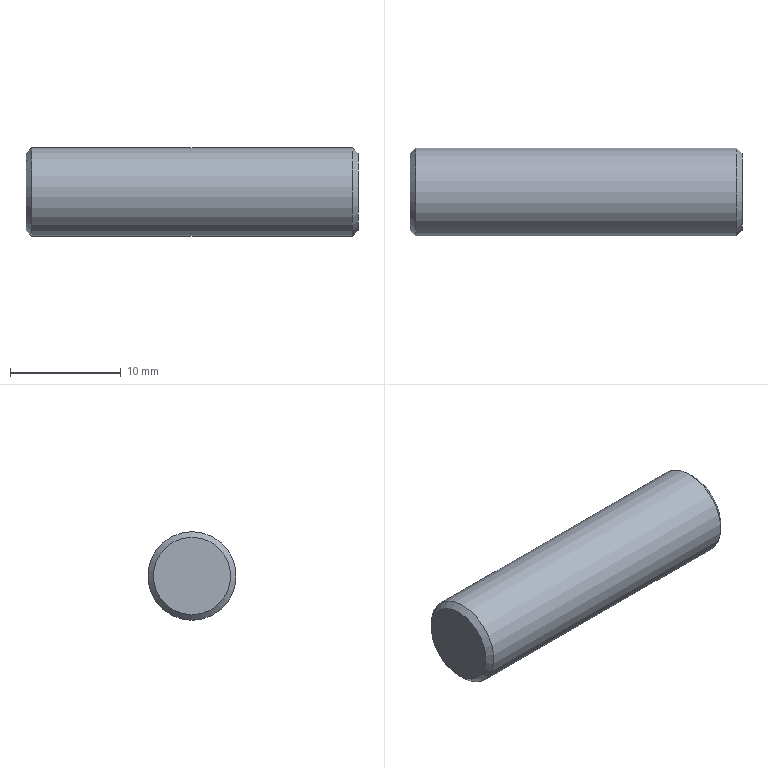Component | NX | DOWEL_PIN_8X30 | 1 solid | 5 faces | box 30 x 8 x 8 mm | volume 1502 mm3 | plane 2 | cone 2 | cylinder 1 | commonest cylinder face diameters 8 x1
STEP:
#1=CARTESIAN_POINT('',(0.,0.,0.));
#2=DIRECTION('',(0.,0.,1.));
#3=DIRECTION('',(1.,0.,0.));
#4=AXIS2_PLACEMENT_3D('',#1,#2,#3);
#5=CARTESIAN_POINT('',(59.511,45.372,16.));
#6=VERTEX_POINT('',#5);
#7=CARTESIAN_POINT('',(59.511,45.372,20.));
#8=DIRECTION('',(-1.,0.,0.));
#9=DIRECTION('',(0.,0.,-1.));
#10=AXIS2_PLACEMENT_3D('',#7,#8,#9);
#11=CIRCLE('',#10,4.);
#12=CARTESIAN_POINT('',(50.011,45.372,20.));
#13=DIRECTION('',(-1.,0.,0.));
#14=DIRECTION('',(0.,0.,1.));
#15=AXIS2_PLACEMENT_3D('',#12,#13,#14);
#16=CYLINDRICAL_SURFACE('',#15,4.);
#17=CARTESIAN_POINT('',(3.142,-9.5));
#18=DIRECTION('',(1.,0.));
#19=VECTOR('',#18,1.);
#20=LINE('',#17,#19);
#21=(GEOMETRIC_REPRESENTATION_CONTEXT(2)PARAMETRIC_REPRESENTATION_CONTEXT()REPRESENTATION_CONTEXT('',''));
#22=DEFINITIONAL_REPRESENTATION('',(#20),#21);
#23=PCURVE('',#16,#22);
#24=CARTESIAN_POINT('',(60.011,45.372,20.));
#25=DIRECTION('',(-1.,0.,0.));
#26=DIRECTION('',(0.,0.,1.));
#27=AXIS2_PLACEMENT_3D('',#24,#25,#26);
#28=CONICAL_SURFACE('',#27,3.5,0.7854);
#29=CARTESIAN_POINT('',(3.142,0.5));
#30=DIRECTION('',(1.,0.));
#31=VECTOR('',#30,1.);
#32=LINE('',#29,#31);
#33=(GEOMETRIC_REPRESENTATION_CONTEXT(2)PARAMETRIC_REPRESENTATION_CONTEXT()REPRESENTATION_CONTEXT('',''));
#34=DEFINITIONAL_REPRESENTATION('',(#32),#33);
#35=PCURVE('',#28,#34);
#36=SURFACE_CURVE('',#11,(#23,#35),.PCURVE_S1.);
#37=EDGE_CURVE('',#6,#6,#36,.T.);
#38=ORIENTED_EDGE('',*,*,#37,.T.);
#39=CARTESIAN_POINT('',(30.511,45.372,16.));
#40=VERTEX_POINT('',#39);
#41=CARTESIAN_POINT('',(59.511,45.372,16.));
#42=CARTESIAN_POINT('',(30.511,45.372,16.));
#43=B_SPLINE_CURVE_WITH_KNOTS('',1,(#41,#42),.UNSPECIFIED.,.F.,.F.,(2,2),(-9.5,19.5),.PIECEWISE_BEZIER_KNOTS.);
#44=CARTESIAN_POINT('',(9.425,0.));
#45=DIRECTION('',(0.,1.));
#46=VECTOR('',#45,1.);
#47=LINE('',#44,#46);
#48=(GEOMETRIC_REPRESENTATION_CONTEXT(2)PARAMETRIC_REPRESENTATION_CONTEXT()REPRESENTATION_CONTEXT('',''));
#49=DEFINITIONAL_REPRESENTATION('',(#47),#48);
#50=PCURVE('',#16,#49);
#51=CARTESIAN_POINT('',(3.142,0.));
#52=DIRECTION('',(0.,1.));
#53=VECTOR('',#52,1.);
#54=LINE('',#51,#53);
#55=(GEOMETRIC_REPRESENTATION_CONTEXT(2)PARAMETRIC_REPRESENTATION_CONTEXT()REPRESENTATION_CONTEXT('',''));
#56=DEFINITIONAL_REPRESENTATION('',(#54),#55);
#57=PCURVE('',#16,#56);
#58=SEAM_CURVE('',#43,(#50,#57),.PCURVE_S1.);
#59=EDGE_CURVE('',#6,#40,#58,.T.);
#60=ORIENTED_EDGE('',*,*,#59,.T.);
#61=CARTESIAN_POINT('',(30.511,45.372,20.));
#62=DIRECTION('',(1.,0.,0.));
#63=DIRECTION('',(0.,0.,-1.));
#64=AXIS2_PLACEMENT_3D('',#61,#62,#63);
#65=CIRCLE('',#64,4.);
#66=CARTESIAN_POINT('',(9.425,19.5));
#67=DIRECTION('',(-1.,0.));
#68=VECTOR('',#67,1.);
#69=LINE('',#66,#68);
#70=(GEOMETRIC_REPRESENTATION_CONTEXT(2)PARAMETRIC_REPRESENTATION_CONTEXT()REPRESENTATION_CONTEXT('',''));
#71=DEFINITIONAL_REPRESENTATION('',(#69),#70);
#72=PCURVE('',#16,#71);
#73=CARTESIAN_POINT('',(30.511,45.372,20.));
#74=DIRECTION('',(1.,0.,0.));
#75=DIRECTION('',(0.,0.,-1.));
#76=AXIS2_PLACEMENT_3D('',#73,#74,#75);
#77=CONICAL_SURFACE('',#76,4.,0.7854);
#78=CARTESIAN_POINT('',(0.,0.));
#79=DIRECTION('',(1.,0.));
#80=VECTOR('',#79,1.);
#81=LINE('',#78,#80);
#82=(GEOMETRIC_REPRESENTATION_CONTEXT(2)PARAMETRIC_REPRESENTATION_CONTEXT()REPRESENTATION_CONTEXT('',''));
#83=DEFINITIONAL_REPRESENTATION('',(#81),#82);
#84=PCURVE('',#77,#83);
#85=SURFACE_CURVE('',#65,(#72,#84),.PCURVE_S1.);
#86=EDGE_CURVE('',#40,#40,#85,.T.);
#87=ORIENTED_EDGE('',*,*,#86,.T.);
#88=ORIENTED_EDGE('',*,*,#59,.F.);
#89=EDGE_LOOP('',(#38,#60,#87,#88));
#90=FACE_BOUND('',#89,.T.);
#91=ADVANCED_FACE('',(#90),#16,.T.);
#92=CARTESIAN_POINT('',(60.011,45.372,16.5));
#93=VERTEX_POINT('',#92);
#94=CARTESIAN_POINT('',(60.011,45.372,20.));
#95=DIRECTION('',(1.,0.,0.));
#96=DIRECTION('',(0.,0.,-1.));
#97=AXIS2_PLACEMENT_3D('',#94,#95,#96);
#98=CIRCLE('',#97,3.5);
#99=CARTESIAN_POINT('',(60.011,45.372,20.));
#100=DIRECTION('',(1.,0.,0.));
#101=DIRECTION('',(0.,0.,-1.));
#102=AXIS2_PLACEMENT_3D('',#99,#100,#101);
#103=PLANE('',#102);
#104=CARTESIAN_POINT('',(0.,0.));
#105=DIRECTION('',(1.,0.));
#106=AXIS2_PLACEMENT_2D('',#104,#105);
#107=CIRCLE('',#106,3.5);
#108=(GEOMETRIC_REPRESENTATION_CONTEXT(2)PARAMETRIC_REPRESENTATION_CONTEXT()REPRESENTATION_CONTEXT('',''));
#109=DEFINITIONAL_REPRESENTATION('',(#107),#108);
#110=PCURVE('',#103,#109);
#111=CARTESIAN_POINT('',(9.425,0.));
#112=DIRECTION('',(-1.,0.));
#113=VECTOR('',#112,1.);
#114=LINE('',#111,#113);
#115=(GEOMETRIC_REPRESENTATION_CONTEXT(2)PARAMETRIC_REPRESENTATION_CONTEXT()REPRESENTATION_CONTEXT('',''));
#116=DEFINITIONAL_REPRESENTATION('',(#114),#115);
#117=PCURVE('',#28,#116);
#118=SURFACE_CURVE('',#98,(#110,#117),.PCURVE_S1.);
#119=EDGE_CURVE('',#93,#93,#118,.T.);
#120=ORIENTED_EDGE('',*,*,#119,.T.);
#121=EDGE_LOOP('',(#120));
#122=FACE_BOUND('',#121,.T.);
#123=ADVANCED_FACE('',(#122),#103,.T.);
#124=CARTESIAN_POINT('',(30.011,45.372,16.5));
#125=VERTEX_POINT('',#124);
#126=CARTESIAN_POINT('',(30.011,45.372,20.));
#127=DIRECTION('',(-1.,0.,0.));
#128=DIRECTION('',(0.,0.,-1.));
#129=AXIS2_PLACEMENT_3D('',#126,#127,#128);
#130=CIRCLE('',#129,3.5);
#131=CARTESIAN_POINT('',(30.011,45.372,20.));
#132=DIRECTION('',(1.,0.,0.));
#133=DIRECTION('',(0.,0.,-1.));
#134=AXIS2_PLACEMENT_3D('',#131,#132,#133);
#135=PLANE('',#134);
#136=CARTESIAN_POINT('',(3.5,0.));
#137=CARTESIAN_POINT('',(3.5,-6.062));
#138=CARTESIAN_POINT('',(-1.75,-3.031));
#139=CARTESIAN_POINT('',(-7.,-0.));
#140=CARTESIAN_POINT('',(-1.75,3.031));
#141=CARTESIAN_POINT('',(3.5,6.062));
#142=CARTESIAN_POINT('',(3.5,0.));
#143=(BOUNDED_CURVE()B_SPLINE_CURVE(2,(#136,#137,#138,#139,#140,#141,#142),.UNSPECIFIED.,.T.,.F.)B_SPLINE_CURVE_WITH_KNOTS((1,2,2,2,2,1),(-2.094,0.,2.094,4.189,6.283,8.378),.UNSPECIFIED.)CURVE()GEOMETRIC_REPRESENTATION_ITEM()RATIONAL_B_SPLINE_CURVE((1.,0.5,1.,0.5,1.,0.5,1.))REPRESENTATION_ITEM(''));
#144=(GEOMETRIC_REPRESENTATION_CONTEXT(2)PARAMETRIC_REPRESENTATION_CONTEXT()REPRESENTATION_CONTEXT('',''));
#145=DEFINITIONAL_REPRESENTATION('',(#143),#144);
#146=PCURVE('',#135,#145);
#147=CARTESIAN_POINT('',(6.283,-0.5));
#148=DIRECTION('',(-1.,0.));
#149=VECTOR('',#148,1.);
#150=LINE('',#147,#149);
#151=(GEOMETRIC_REPRESENTATION_CONTEXT(2)PARAMETRIC_REPRESENTATION_CONTEXT()REPRESENTATION_CONTEXT('',''));
#152=DEFINITIONAL_REPRESENTATION('',(#150),#151);
#153=PCURVE('',#77,#152);
#154=SURFACE_CURVE('',#130,(#146,#153),.PCURVE_S1.);
#155=EDGE_CURVE('',#125,#125,#154,.T.);
#156=ORIENTED_EDGE('',*,*,#155,.T.);
#157=EDGE_LOOP('',(#156));
#158=FACE_BOUND('',#157,.T.);
#159=ADVANCED_FACE('',(#158),#135,.F.);
#160=ORIENTED_EDGE('',*,*,#37,.F.);
#161=CARTESIAN_POINT('',(60.011,45.372,16.5));
#162=CARTESIAN_POINT('',(59.511,45.372,16.));
#163=B_SPLINE_CURVE_WITH_KNOTS('',1,(#161,#162),.UNSPECIFIED.,.F.,.F.,(2,2),(0.,0.7071),.PIECEWISE_BEZIER_KNOTS.);
#164=CARTESIAN_POINT('',(3.142,0.));
#165=DIRECTION('',(0.,1.));
#166=VECTOR('',#165,1.);
#167=LINE('',#164,#166);
#168=(GEOMETRIC_REPRESENTATION_CONTEXT(2)PARAMETRIC_REPRESENTATION_CONTEXT()REPRESENTATION_CONTEXT('',''));
#169=DEFINITIONAL_REPRESENTATION('',(#167),#168);
#170=PCURVE('',#28,#169);
#171=CARTESIAN_POINT('',(9.425,0.));
#172=DIRECTION('',(0.,1.));
#173=VECTOR('',#172,1.);
#174=LINE('',#171,#173);
#175=(GEOMETRIC_REPRESENTATION_CONTEXT(2)PARAMETRIC_REPRESENTATION_CONTEXT()REPRESENTATION_CONTEXT('',''));
#176=DEFINITIONAL_REPRESENTATION('',(#174),#175);
#177=PCURVE('',#28,#176);
#178=SEAM_CURVE('',#163,(#170,#177),.PCURVE_S1.);
#179=EDGE_CURVE('',#93,#6,#178,.T.);
#180=ORIENTED_EDGE('',*,*,#179,.F.);
#181=ORIENTED_EDGE('',*,*,#119,.F.);
#182=ORIENTED_EDGE('',*,*,#179,.T.);
#183=EDGE_LOOP('',(#160,#180,#181,#182));
#184=FACE_BOUND('',#183,.T.);
#185=ADVANCED_FACE('',(#184),#28,.T.);
#186=ORIENTED_EDGE('',*,*,#155,.F.);
#187=CARTESIAN_POINT('',(30.011,45.372,16.5));
#188=CARTESIAN_POINT('',(30.511,45.372,16.));
#189=B_SPLINE_CURVE_WITH_KNOTS('',1,(#187,#188),.UNSPECIFIED.,.F.,.F.,(2,2),(-0.7071,0.),.PIECEWISE_BEZIER_KNOTS.);
#190=CARTESIAN_POINT('',(6.283,0.));
#191=DIRECTION('',(0.,1.));
#192=VECTOR('',#191,1.);
#193=LINE('',#190,#192);
#194=(GEOMETRIC_REPRESENTATION_CONTEXT(2)PARAMETRIC_REPRESENTATION_CONTEXT()REPRESENTATION_CONTEXT('',''));
#195=DEFINITIONAL_REPRESENTATION('',(#193),#194);
#196=PCURVE('',#77,#195);
#197=CARTESIAN_POINT('',(0.,0.));
#198=DIRECTION('',(0.,1.));
#199=VECTOR('',#198,1.);
#200=LINE('',#197,#199);
#201=(GEOMETRIC_REPRESENTATION_CONTEXT(2)PARAMETRIC_REPRESENTATION_CONTEXT()REPRESENTATION_CONTEXT('',''));
#202=DEFINITIONAL_REPRESENTATION('',(#200),#201);
#203=PCURVE('',#77,#202);
#204=SEAM_CURVE('',#189,(#196,#203),.PCURVE_S1.);
#205=EDGE_CURVE('',#125,#40,#204,.T.);
#206=ORIENTED_EDGE('',*,*,#205,.T.);
#207=ORIENTED_EDGE('',*,*,#86,.F.);
#208=ORIENTED_EDGE('',*,*,#205,.F.);
#209=EDGE_LOOP('',(#186,#206,#207,#208));
#210=FACE_BOUND('',#209,.T.);
#211=ADVANCED_FACE('',(#210),#77,.T.);
#212=CLOSED_SHELL('',(#91,#123,#159,#185,#211));
#213=MANIFOLD_SOLID_BREP('',#212);
#214=(LENGTH_UNIT()NAMED_UNIT(*)SI_UNIT(.MILLI.,.METRE.));
#215=UNCERTAINTY_MEASURE_WITH_UNIT(LENGTH_MEASURE(0.00001),#214,'','');
#216=(NAMED_UNIT(*)PLANE_ANGLE_UNIT()SI_UNIT($,.RADIAN.));
#217=(NAMED_UNIT(*)SI_UNIT($,.STERADIAN.)SOLID_ANGLE_UNIT());
#218=(GEOMETRIC_REPRESENTATION_CONTEXT(3)GLOBAL_UNCERTAINTY_ASSIGNED_CONTEXT((#215))GLOBAL_UNIT_ASSIGNED_CONTEXT((#214,#216,#217))REPRESENTATION_CONTEXT('',''));
#219=ADVANCED_BREP_SHAPE_REPRESENTATION('',(#4,#213),#218);